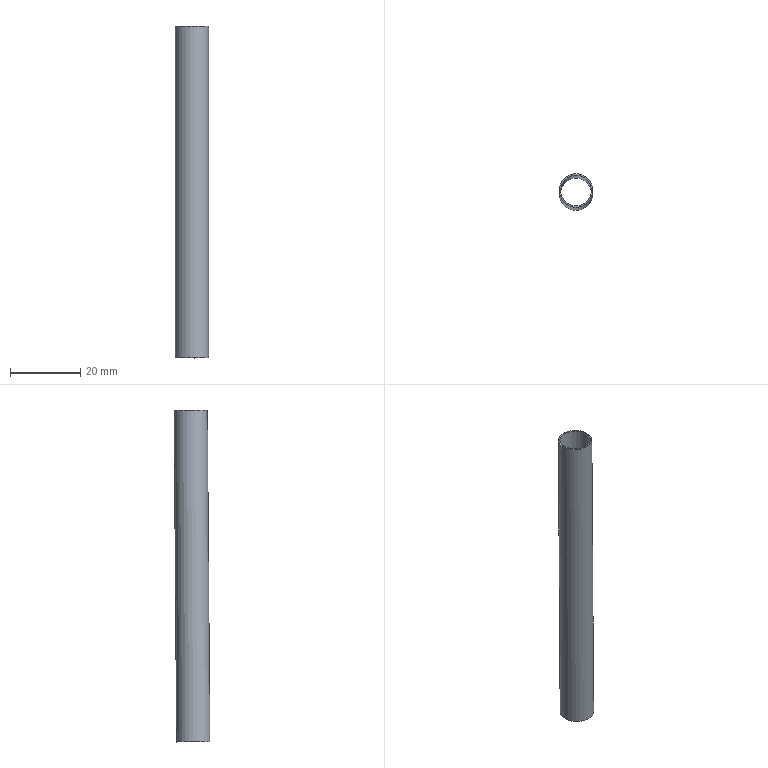Component | NX | TUBE_2 | 1 solid | 4 faces | box 9.53 x 10.24 x 94.32 mm | volume 1081 mm3 | plane 2 | cylinder 2 | commonest cylinder face diameters 9.525 x1 8.725 x1
STEP:
#1=CARTESIAN_POINT('',(0.,0.,0.));
#2=DIRECTION('',(0.,0.,1.));
#3=DIRECTION('',(1.,0.,0.));
#4=AXIS2_PLACEMENT_3D('',#1,#2,#3);
#5=CARTESIAN_POINT('',(51.584,-45.075,158.058));
#6=VERTEX_POINT('',#5);
#7=CARTESIAN_POINT('',(47.221,-45.075,158.058));
#8=DIRECTION('',(-0.0000015,-0.007573,-1.));
#9=DIRECTION('',(1.,0.00009493,-0.00000222));
#10=AXIS2_PLACEMENT_3D('',#7,#8,#9);
#11=CIRCLE('',#10,4.362);
#12=CARTESIAN_POINT('',(47.221,-45.075,158.058));
#13=DIRECTION('',(0.0000015,0.007573,1.));
#14=DIRECTION('',(1.,0.00009493,-0.00000222));
#15=AXIS2_PLACEMENT_3D('',#12,#13,#14);
#16=PLANE('',#15);
#17=CARTESIAN_POINT('',(4.362,-0.));
#18=CARTESIAN_POINT('',(4.362,-7.556));
#19=CARTESIAN_POINT('',(-2.181,-3.778));
#20=CARTESIAN_POINT('',(-8.725,0.));
#21=CARTESIAN_POINT('',(-2.181,3.778));
#22=CARTESIAN_POINT('',(4.362,7.556));
#23=CARTESIAN_POINT('',(4.362,-0.));
#24=(BOUNDED_CURVE()B_SPLINE_CURVE(2,(#17,#18,#19,#20,#21,#22,#23),.UNSPECIFIED.,.T.,.F.)B_SPLINE_CURVE_WITH_KNOTS((1,2,2,2,2,1),(-2.094,0.,2.094,4.189,6.283,8.378),.UNSPECIFIED.)CURVE()GEOMETRIC_REPRESENTATION_ITEM()RATIONAL_B_SPLINE_CURVE((1.,0.5,1.,0.5,1.,0.5,1.))REPRESENTATION_ITEM(''));
#25=(GEOMETRIC_REPRESENTATION_CONTEXT(2)PARAMETRIC_REPRESENTATION_CONTEXT()REPRESENTATION_CONTEXT('',''));
#26=DEFINITIONAL_REPRESENTATION('',(#24),#25);
#27=PCURVE('',#16,#26);
#28=CARTESIAN_POINT('',(47.221,-45.789,63.811));
#29=DIRECTION('',(0.0000015,0.007573,1.));
#30=DIRECTION('',(1.,0.00009493,-0.00000222));
#31=AXIS2_PLACEMENT_3D('',#28,#29,#30);
#32=CYLINDRICAL_SURFACE('',#31,4.362);
#33=CARTESIAN_POINT('',(6.283,94.25));
#34=DIRECTION('',(-1.,0.));
#35=VECTOR('',#34,1.);
#36=LINE('',#33,#35);
#37=(GEOMETRIC_REPRESENTATION_CONTEXT(2)PARAMETRIC_REPRESENTATION_CONTEXT()REPRESENTATION_CONTEXT('',''));
#38=DEFINITIONAL_REPRESENTATION('',(#36),#37);
#39=PCURVE('',#32,#38);
#40=SURFACE_CURVE('',#11,(#27,#39),.PCURVE_S1.);
#41=EDGE_CURVE('',#6,#6,#40,.T.);
#42=ORIENTED_EDGE('',*,*,#41,.T.);
#43=EDGE_LOOP('',(#42));
#44=FACE_BOUND('',#43,.T.);
#45=CARTESIAN_POINT('',(51.984,-45.075,158.058));
#46=VERTEX_POINT('',#45);
#47=CARTESIAN_POINT('',(47.221,-45.075,158.058));
#48=DIRECTION('',(-0.0000015,-0.007573,-1.));
#49=DIRECTION('',(1.,0.00009493,-0.00000222));
#50=AXIS2_PLACEMENT_3D('',#47,#48,#49);
#51=CIRCLE('',#50,4.763);
#52=CARTESIAN_POINT('',(4.763,-0.));
#53=CARTESIAN_POINT('',(4.763,-8.249));
#54=CARTESIAN_POINT('',(-2.381,-4.124));
#55=CARTESIAN_POINT('',(-9.525,0.));
#56=CARTESIAN_POINT('',(-2.381,4.124));
#57=CARTESIAN_POINT('',(4.763,8.249));
#58=CARTESIAN_POINT('',(4.763,-0.));
#59=(BOUNDED_CURVE()B_SPLINE_CURVE(2,(#52,#53,#54,#55,#56,#57,#58),.UNSPECIFIED.,.T.,.F.)B_SPLINE_CURVE_WITH_KNOTS((1,2,2,2,2,1),(-2.094,0.,2.094,4.189,6.283,8.378),.UNSPECIFIED.)CURVE()GEOMETRIC_REPRESENTATION_ITEM()RATIONAL_B_SPLINE_CURVE((1.,0.5,1.,0.5,1.,0.5,1.))REPRESENTATION_ITEM(''));
#60=(GEOMETRIC_REPRESENTATION_CONTEXT(2)PARAMETRIC_REPRESENTATION_CONTEXT()REPRESENTATION_CONTEXT('',''));
#61=DEFINITIONAL_REPRESENTATION('',(#59),#60);
#62=PCURVE('',#16,#61);
#63=CARTESIAN_POINT('',(47.221,-45.789,63.811));
#64=DIRECTION('',(0.0000015,0.007573,1.));
#65=DIRECTION('',(1.,0.00009493,-0.00000222));
#66=AXIS2_PLACEMENT_3D('',#63,#64,#65);
#67=CYLINDRICAL_SURFACE('',#66,4.763);
#68=CARTESIAN_POINT('',(6.283,94.25));
#69=DIRECTION('',(-1.,0.));
#70=VECTOR('',#69,1.);
#71=LINE('',#68,#70);
#72=(GEOMETRIC_REPRESENTATION_CONTEXT(2)PARAMETRIC_REPRESENTATION_CONTEXT()REPRESENTATION_CONTEXT('',''));
#73=DEFINITIONAL_REPRESENTATION('',(#71),#72);
#74=PCURVE('',#67,#73);
#75=SURFACE_CURVE('',#51,(#62,#74),.PCURVE_S1.);
#76=EDGE_CURVE('',#46,#46,#75,.T.);
#77=ORIENTED_EDGE('',*,*,#76,.F.);
#78=EDGE_LOOP('',(#77));
#79=FACE_BOUND('',#78,.T.);
#80=ADVANCED_FACE('',(#44,#79),#16,.T.);
#81=CARTESIAN_POINT('',(42.859,-45.789,63.811));
#82=VERTEX_POINT('',#81);
#83=CARTESIAN_POINT('',(51.584,-45.789,63.811));
#84=VERTEX_POINT('',#83);
#85=CARTESIAN_POINT('',(47.221,-45.789,63.811));
#86=DIRECTION('',(0.0000015,0.007573,1.));
#87=DIRECTION('',(-1.,-0.00009493,0.00000222));
#88=AXIS2_PLACEMENT_3D('',#85,#86,#87);
#89=CIRCLE('',#88,4.362);
#90=CARTESIAN_POINT('',(47.221,-45.789,63.811));
#91=DIRECTION('',(-0.0000015,-0.007573,-1.));
#92=DIRECTION('',(-1.,-0.00009493,0.00000222));
#93=AXIS2_PLACEMENT_3D('',#90,#91,#92);
#94=PLANE('',#93);
#95=CARTESIAN_POINT('',(4.362,0.));
#96=CARTESIAN_POINT('',(4.362,-7.556));
#97=CARTESIAN_POINT('',(-2.181,-3.778));
#98=CARTESIAN_POINT('',(-8.725,-0.));
#99=CARTESIAN_POINT('',(-2.181,3.778));
#100=CARTESIAN_POINT('',(4.362,7.556));
#101=CARTESIAN_POINT('',(4.362,0.));
#102=(BOUNDED_CURVE()B_SPLINE_CURVE(2,(#95,#96,#97,#98,#99,#100,#101),.UNSPECIFIED.,.T.,.F.)B_SPLINE_CURVE_WITH_KNOTS((1,2,2,2,2,1),(-2.094,0.,2.094,4.189,6.283,8.378),.UNSPECIFIED.)CURVE()GEOMETRIC_REPRESENTATION_ITEM()RATIONAL_B_SPLINE_CURVE((1.,0.5,1.,0.5,1.,0.5,1.))REPRESENTATION_ITEM(''));
#103=(GEOMETRIC_REPRESENTATION_CONTEXT(2)PARAMETRIC_REPRESENTATION_CONTEXT()REPRESENTATION_CONTEXT('',''));
#104=DEFINITIONAL_REPRESENTATION('',(#102),#103);
#105=PCURVE('',#94,#104);
#106=CARTESIAN_POINT('',(3.142,0.));
#107=DIRECTION('',(1.,0.));
#108=VECTOR('',#107,1.);
#109=LINE('',#106,#108);
#110=(GEOMETRIC_REPRESENTATION_CONTEXT(2)PARAMETRIC_REPRESENTATION_CONTEXT()REPRESENTATION_CONTEXT('',''));
#111=DEFINITIONAL_REPRESENTATION('',(#109),#110);
#112=PCURVE('',#32,#111);
#113=SURFACE_CURVE('',#89,(#105,#112),.PCURVE_S1.);
#114=EDGE_CURVE('',#82,#84,#113,.T.);
#115=ORIENTED_EDGE('',*,*,#114,.T.);
#116=CARTESIAN_POINT('',(47.221,-45.789,63.811));
#117=DIRECTION('',(0.0000015,0.007573,1.));
#118=DIRECTION('',(-1.,-0.00009493,0.00000222));
#119=AXIS2_PLACEMENT_3D('',#116,#117,#118);
#120=CIRCLE('',#119,4.362);
#121=CARTESIAN_POINT('',(4.362,0.));
#122=CARTESIAN_POINT('',(4.362,-7.556));
#123=CARTESIAN_POINT('',(-2.181,-3.778));
#124=CARTESIAN_POINT('',(-8.725,-0.));
#125=CARTESIAN_POINT('',(-2.181,3.778));
#126=CARTESIAN_POINT('',(4.362,7.556));
#127=CARTESIAN_POINT('',(4.362,0.));
#128=(BOUNDED_CURVE()B_SPLINE_CURVE(2,(#121,#122,#123,#124,#125,#126,#127),.UNSPECIFIED.,.T.,.F.)B_SPLINE_CURVE_WITH_KNOTS((1,2,2,2,2,1),(-2.094,0.,2.094,4.189,6.283,8.378),.UNSPECIFIED.)CURVE()GEOMETRIC_REPRESENTATION_ITEM()RATIONAL_B_SPLINE_CURVE((1.,0.5,1.,0.5,1.,0.5,1.))REPRESENTATION_ITEM(''));
#129=(GEOMETRIC_REPRESENTATION_CONTEXT(2)PARAMETRIC_REPRESENTATION_CONTEXT()REPRESENTATION_CONTEXT('',''));
#130=DEFINITIONAL_REPRESENTATION('',(#128),#129);
#131=PCURVE('',#94,#130);
#132=CARTESIAN_POINT('',(-3.142,0.));
#133=DIRECTION('',(1.,0.));
#134=VECTOR('',#133,1.);
#135=LINE('',#132,#134);
#136=(GEOMETRIC_REPRESENTATION_CONTEXT(2)PARAMETRIC_REPRESENTATION_CONTEXT()REPRESENTATION_CONTEXT('',''));
#137=DEFINITIONAL_REPRESENTATION('',(#135),#136);
#138=PCURVE('',#32,#137);
#139=SURFACE_CURVE('',#120,(#131,#138),.PCURVE_S1.);
#140=EDGE_CURVE('',#84,#82,#139,.T.);
#141=ORIENTED_EDGE('',*,*,#140,.T.);
#142=EDGE_LOOP('',(#115,#141));
#143=FACE_BOUND('',#142,.T.);
#144=CARTESIAN_POINT('',(51.984,-45.789,63.811));
#145=VERTEX_POINT('',#144);
#146=CARTESIAN_POINT('',(47.221,-45.789,63.811));
#147=DIRECTION('',(0.0000015,0.007573,1.));
#148=DIRECTION('',(1.,0.00009493,-0.00000222));
#149=AXIS2_PLACEMENT_3D('',#146,#147,#148);
#150=CIRCLE('',#149,4.763);
#151=CARTESIAN_POINT('',(-4.763,-0.));
#152=CARTESIAN_POINT('',(-4.763,8.249));
#153=CARTESIAN_POINT('',(2.381,4.124));
#154=CARTESIAN_POINT('',(9.525,0.));
#155=CARTESIAN_POINT('',(2.381,-4.124));
#156=CARTESIAN_POINT('',(-4.763,-8.249));
#157=CARTESIAN_POINT('',(-4.763,-0.));
#158=(BOUNDED_CURVE()B_SPLINE_CURVE(2,(#151,#152,#153,#154,#155,#156,#157),.UNSPECIFIED.,.T.,.F.)B_SPLINE_CURVE_WITH_KNOTS((1,2,2,2,2,1),(-2.094,0.,2.094,4.189,6.283,8.378),.UNSPECIFIED.)CURVE()GEOMETRIC_REPRESENTATION_ITEM()RATIONAL_B_SPLINE_CURVE((1.,0.5,1.,0.5,1.,0.5,1.))REPRESENTATION_ITEM(''));
#159=(GEOMETRIC_REPRESENTATION_CONTEXT(2)PARAMETRIC_REPRESENTATION_CONTEXT()REPRESENTATION_CONTEXT('',''));
#160=DEFINITIONAL_REPRESENTATION('',(#158),#159);
#161=PCURVE('',#94,#160);
#162=CARTESIAN_POINT('',(0.,0.));
#163=DIRECTION('',(1.,0.));
#164=VECTOR('',#163,1.);
#165=LINE('',#162,#164);
#166=(GEOMETRIC_REPRESENTATION_CONTEXT(2)PARAMETRIC_REPRESENTATION_CONTEXT()REPRESENTATION_CONTEXT('',''));
#167=DEFINITIONAL_REPRESENTATION('',(#165),#166);
#168=PCURVE('',#67,#167);
#169=SURFACE_CURVE('',#150,(#161,#168),.PCURVE_S1.);
#170=EDGE_CURVE('',#145,#145,#169,.T.);
#171=ORIENTED_EDGE('',*,*,#170,.F.);
#172=EDGE_LOOP('',(#171));
#173=FACE_BOUND('',#172,.T.);
#174=ADVANCED_FACE('',(#143,#173),#94,.T.);
#175=ORIENTED_EDGE('',*,*,#76,.T.);
#176=CARTESIAN_POINT('',(51.984,-45.789,63.811));
#177=CARTESIAN_POINT('',(51.984,-45.075,158.058));
#178=B_SPLINE_CURVE_WITH_KNOTS('',1,(#176,#177),.UNSPECIFIED.,.F.,.F.,(2,2),(0.,94.25),.PIECEWISE_BEZIER_KNOTS.);
#179=CARTESIAN_POINT('',(0.,0.));
#180=DIRECTION('',(0.,1.));
#181=VECTOR('',#180,1.);
#182=LINE('',#179,#181);
#183=(GEOMETRIC_REPRESENTATION_CONTEXT(2)PARAMETRIC_REPRESENTATION_CONTEXT()REPRESENTATION_CONTEXT('',''));
#184=DEFINITIONAL_REPRESENTATION('',(#182),#183);
#185=PCURVE('',#67,#184);
#186=CARTESIAN_POINT('',(6.283,0.));
#187=DIRECTION('',(0.,1.));
#188=VECTOR('',#187,1.);
#189=LINE('',#186,#188);
#190=(GEOMETRIC_REPRESENTATION_CONTEXT(2)PARAMETRIC_REPRESENTATION_CONTEXT()REPRESENTATION_CONTEXT('',''));
#191=DEFINITIONAL_REPRESENTATION('',(#189),#190);
#192=PCURVE('',#67,#191);
#193=SEAM_CURVE('',#178,(#185,#192),.PCURVE_S1.);
#194=EDGE_CURVE('',#145,#46,#193,.T.);
#195=ORIENTED_EDGE('',*,*,#194,.F.);
#196=ORIENTED_EDGE('',*,*,#170,.T.);
#197=ORIENTED_EDGE('',*,*,#194,.T.);
#198=EDGE_LOOP('',(#175,#195,#196,#197));
#199=FACE_BOUND('',#198,.T.);
#200=ADVANCED_FACE('',(#199),#67,.T.);
#201=ORIENTED_EDGE('',*,*,#41,.T.);
#202=CARTESIAN_POINT('',(51.584,-45.789,63.811));
#203=CARTESIAN_POINT('',(51.584,-45.075,158.058));
#204=B_SPLINE_CURVE_WITH_KNOTS('',1,(#202,#203),.UNSPECIFIED.,.F.,.F.,(2,2),(0.,94.25),.PIECEWISE_BEZIER_KNOTS.);
#205=CARTESIAN_POINT('',(0.,0.));
#206=DIRECTION('',(0.,1.));
#207=VECTOR('',#206,1.);
#208=LINE('',#205,#207);
#209=(GEOMETRIC_REPRESENTATION_CONTEXT(2)PARAMETRIC_REPRESENTATION_CONTEXT()REPRESENTATION_CONTEXT('',''));
#210=DEFINITIONAL_REPRESENTATION('',(#208),#209);
#211=PCURVE('',#32,#210);
#212=CARTESIAN_POINT('',(6.283,0.));
#213=DIRECTION('',(0.,1.));
#214=VECTOR('',#213,1.);
#215=LINE('',#212,#214);
#216=(GEOMETRIC_REPRESENTATION_CONTEXT(2)PARAMETRIC_REPRESENTATION_CONTEXT()REPRESENTATION_CONTEXT('',''));
#217=DEFINITIONAL_REPRESENTATION('',(#215),#216);
#218=PCURVE('',#32,#217);
#219=SEAM_CURVE('',#204,(#211,#218),.PCURVE_S1.);
#220=EDGE_CURVE('',#84,#6,#219,.T.);
#221=ORIENTED_EDGE('',*,*,#220,.F.);
#222=ORIENTED_EDGE('',*,*,#140,.T.);
#223=ORIENTED_EDGE('',*,*,#114,.T.);
#224=ORIENTED_EDGE('',*,*,#220,.T.);
#225=EDGE_LOOP('',(#201,#221,#222,#223,#224));
#226=FACE_BOUND('',#225,.F.);
#227=ADVANCED_FACE('',(#226),#32,.F.);
#228=CLOSED_SHELL('',(#80,#174,#200,#227));
#229=MANIFOLD_SOLID_BREP('',#228);
#230=(LENGTH_UNIT()NAMED_UNIT(*)SI_UNIT(.MILLI.,.METRE.));
#231=UNCERTAINTY_MEASURE_WITH_UNIT(LENGTH_MEASURE(0.000005),#230,'','');
#232=(NAMED_UNIT(*)PLANE_ANGLE_UNIT()SI_UNIT($,.RADIAN.));
#233=(NAMED_UNIT(*)SI_UNIT($,.STERADIAN.)SOLID_ANGLE_UNIT());
#234=(GEOMETRIC_REPRESENTATION_CONTEXT(3)GLOBAL_UNCERTAINTY_ASSIGNED_CONTEXT((#231))GLOBAL_UNIT_ASSIGNED_CONTEXT((#230,#232,#233))REPRESENTATION_CONTEXT('',''));
#235=ADVANCED_BREP_SHAPE_REPRESENTATION('',(#4,#229),#234);